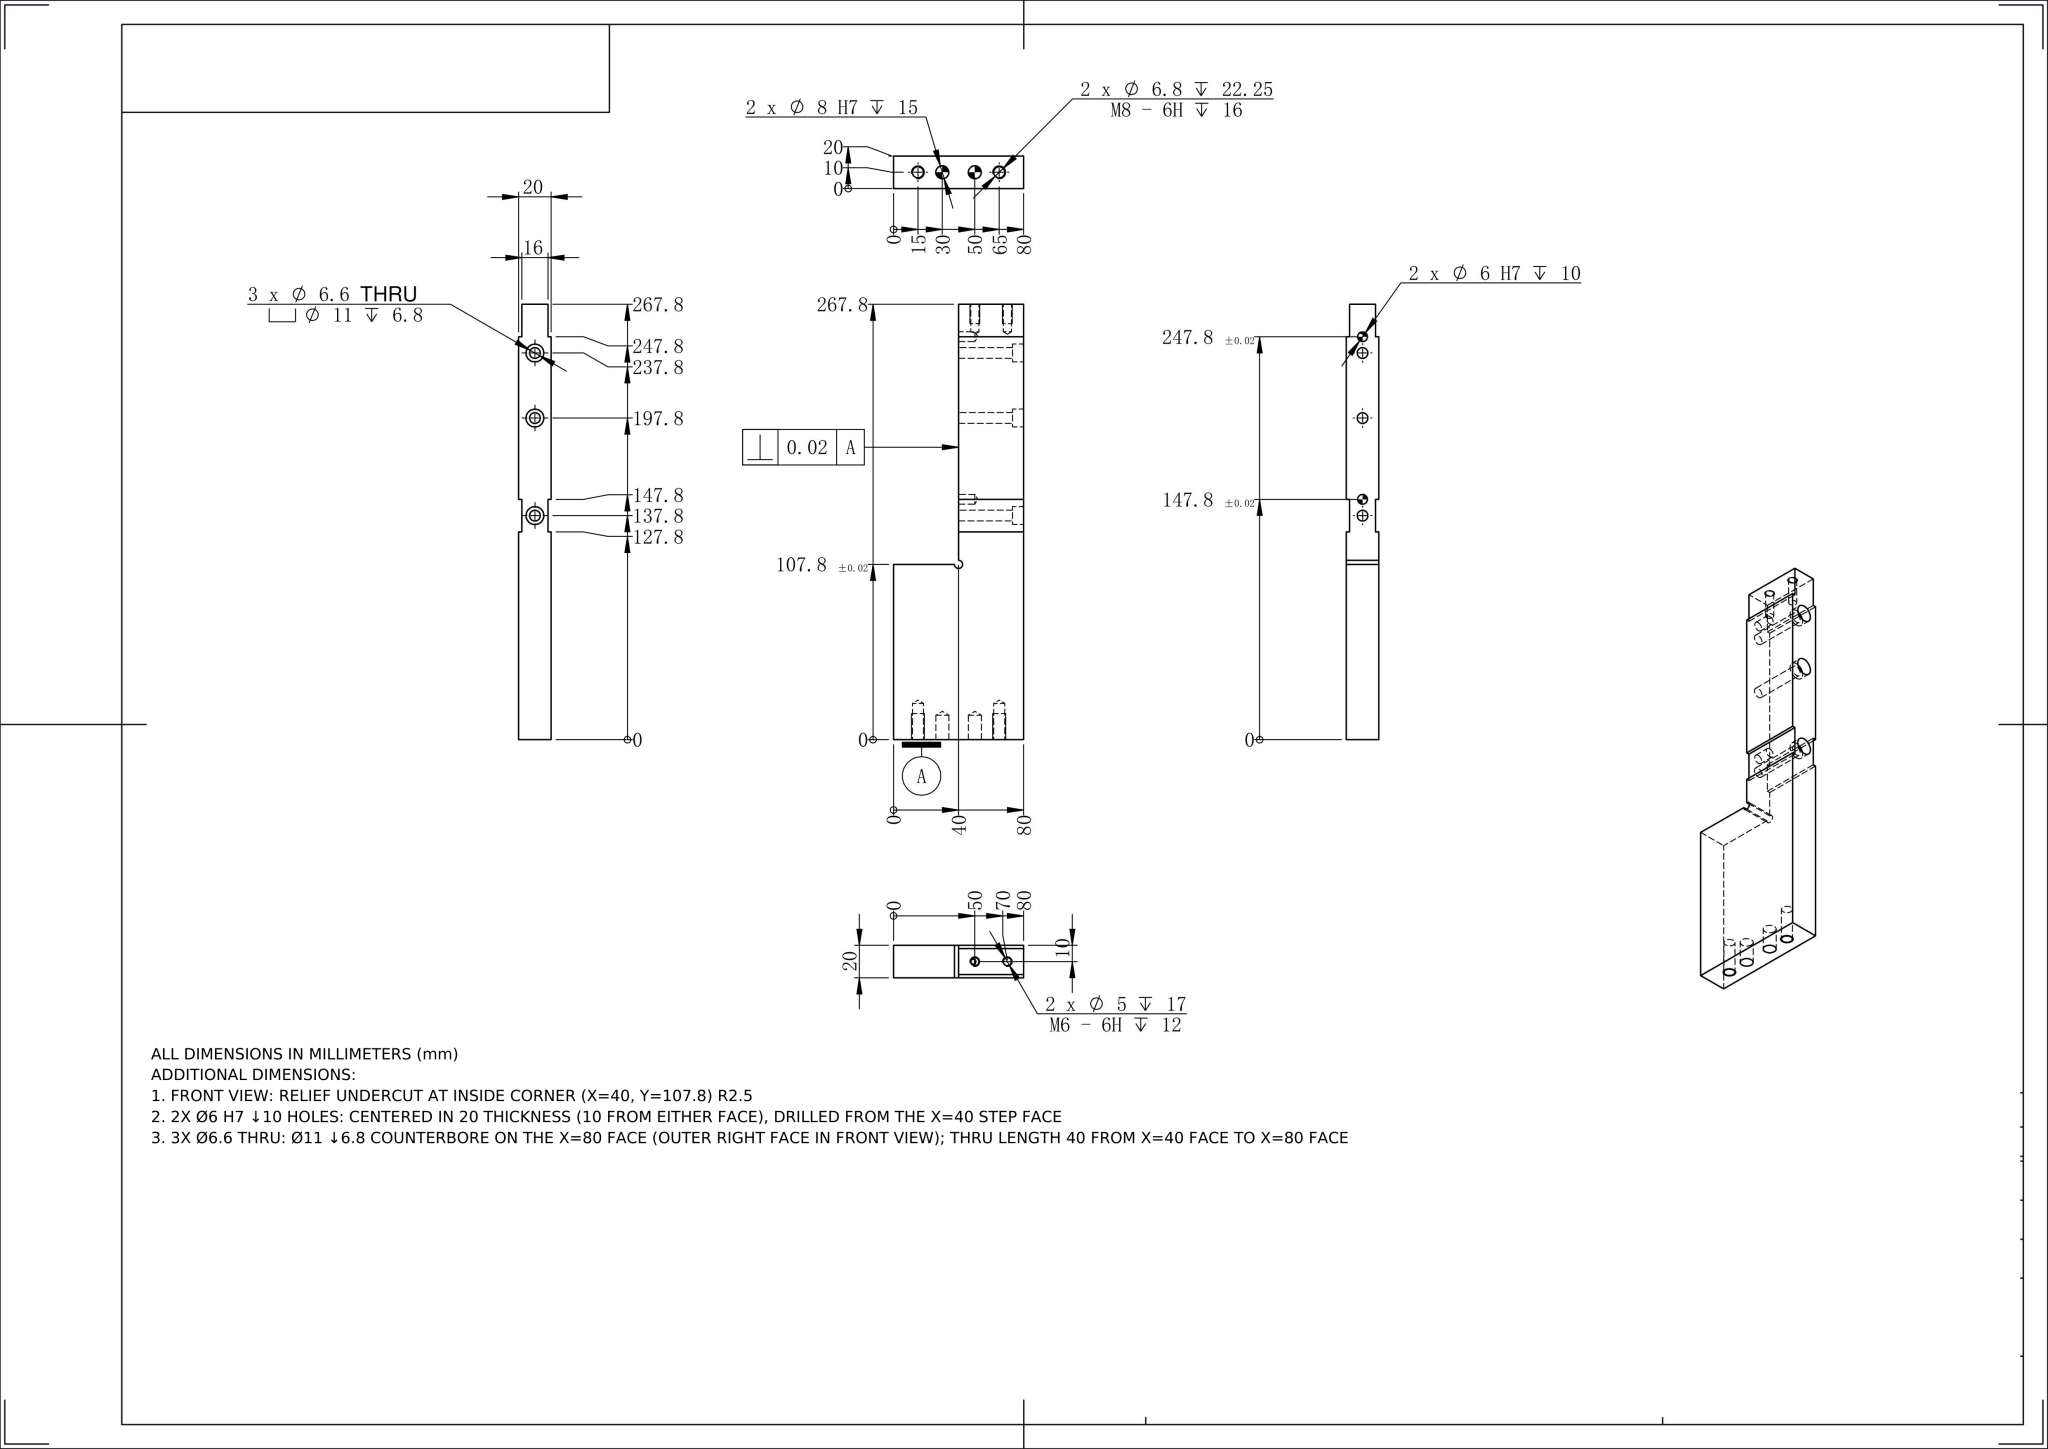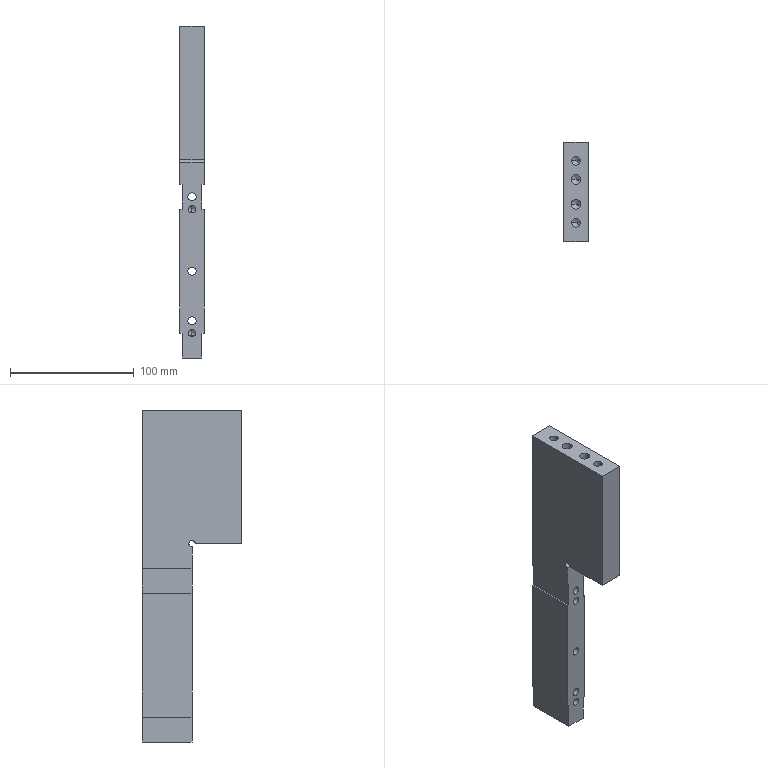Part | NX | mm | 1 solid | 69 faces | box 20 x 80 x 267.8 mm | volume 283903 mm3 | cylinder 30 | plane 23 | cone 16 | commonest cylinder face diameters 5 x6 11 x6 6.6 x6 8 x4 6.8 x4 6 x4